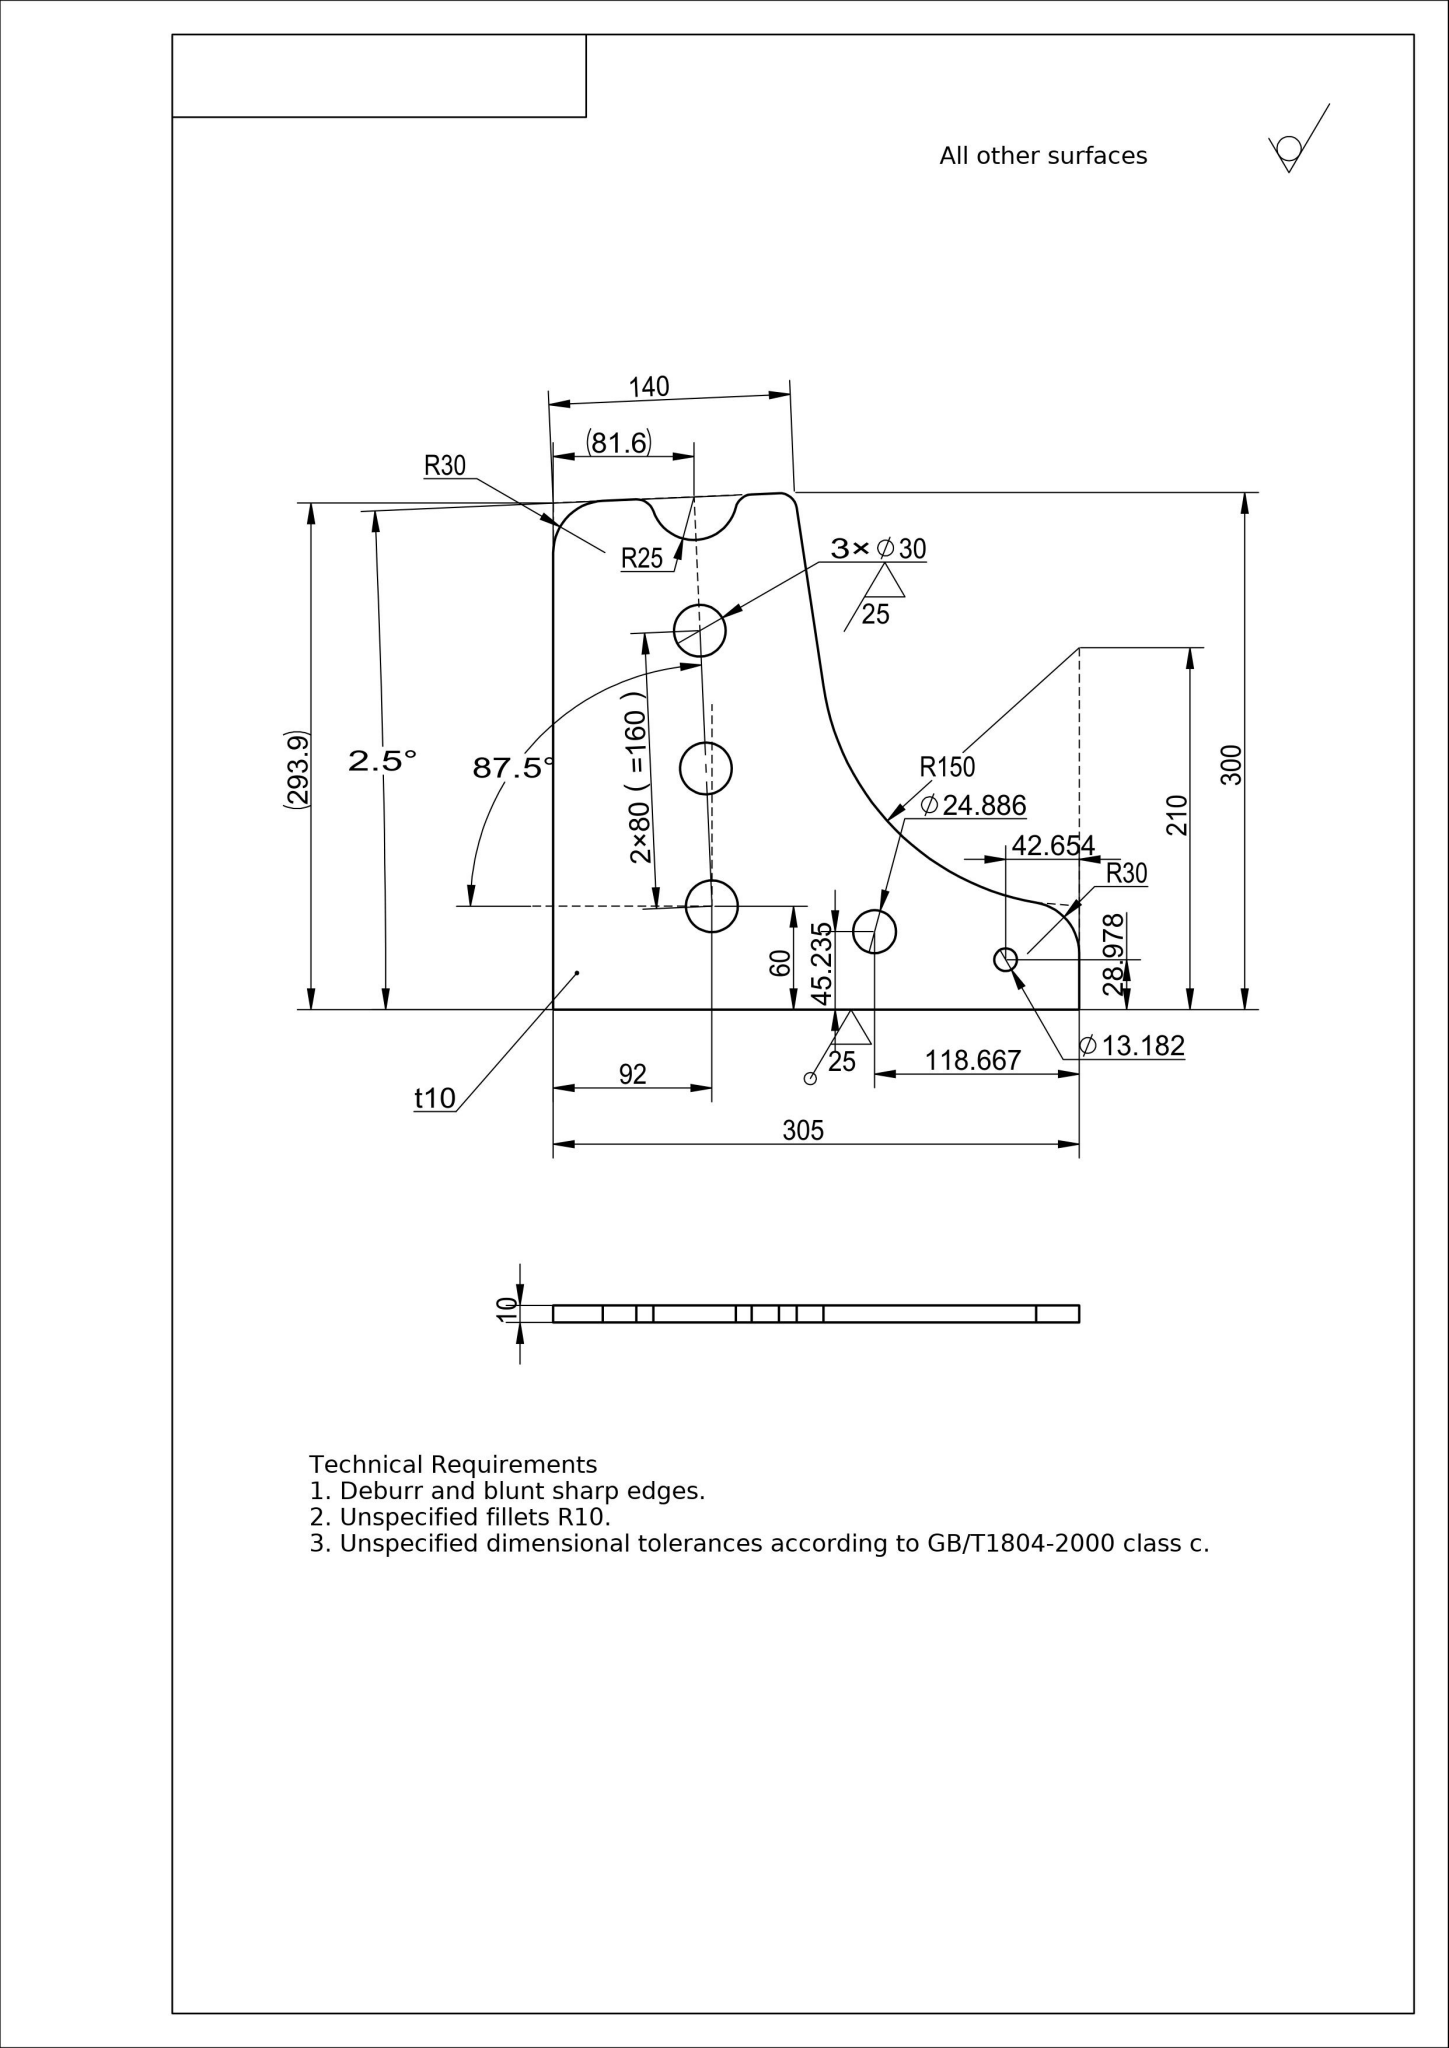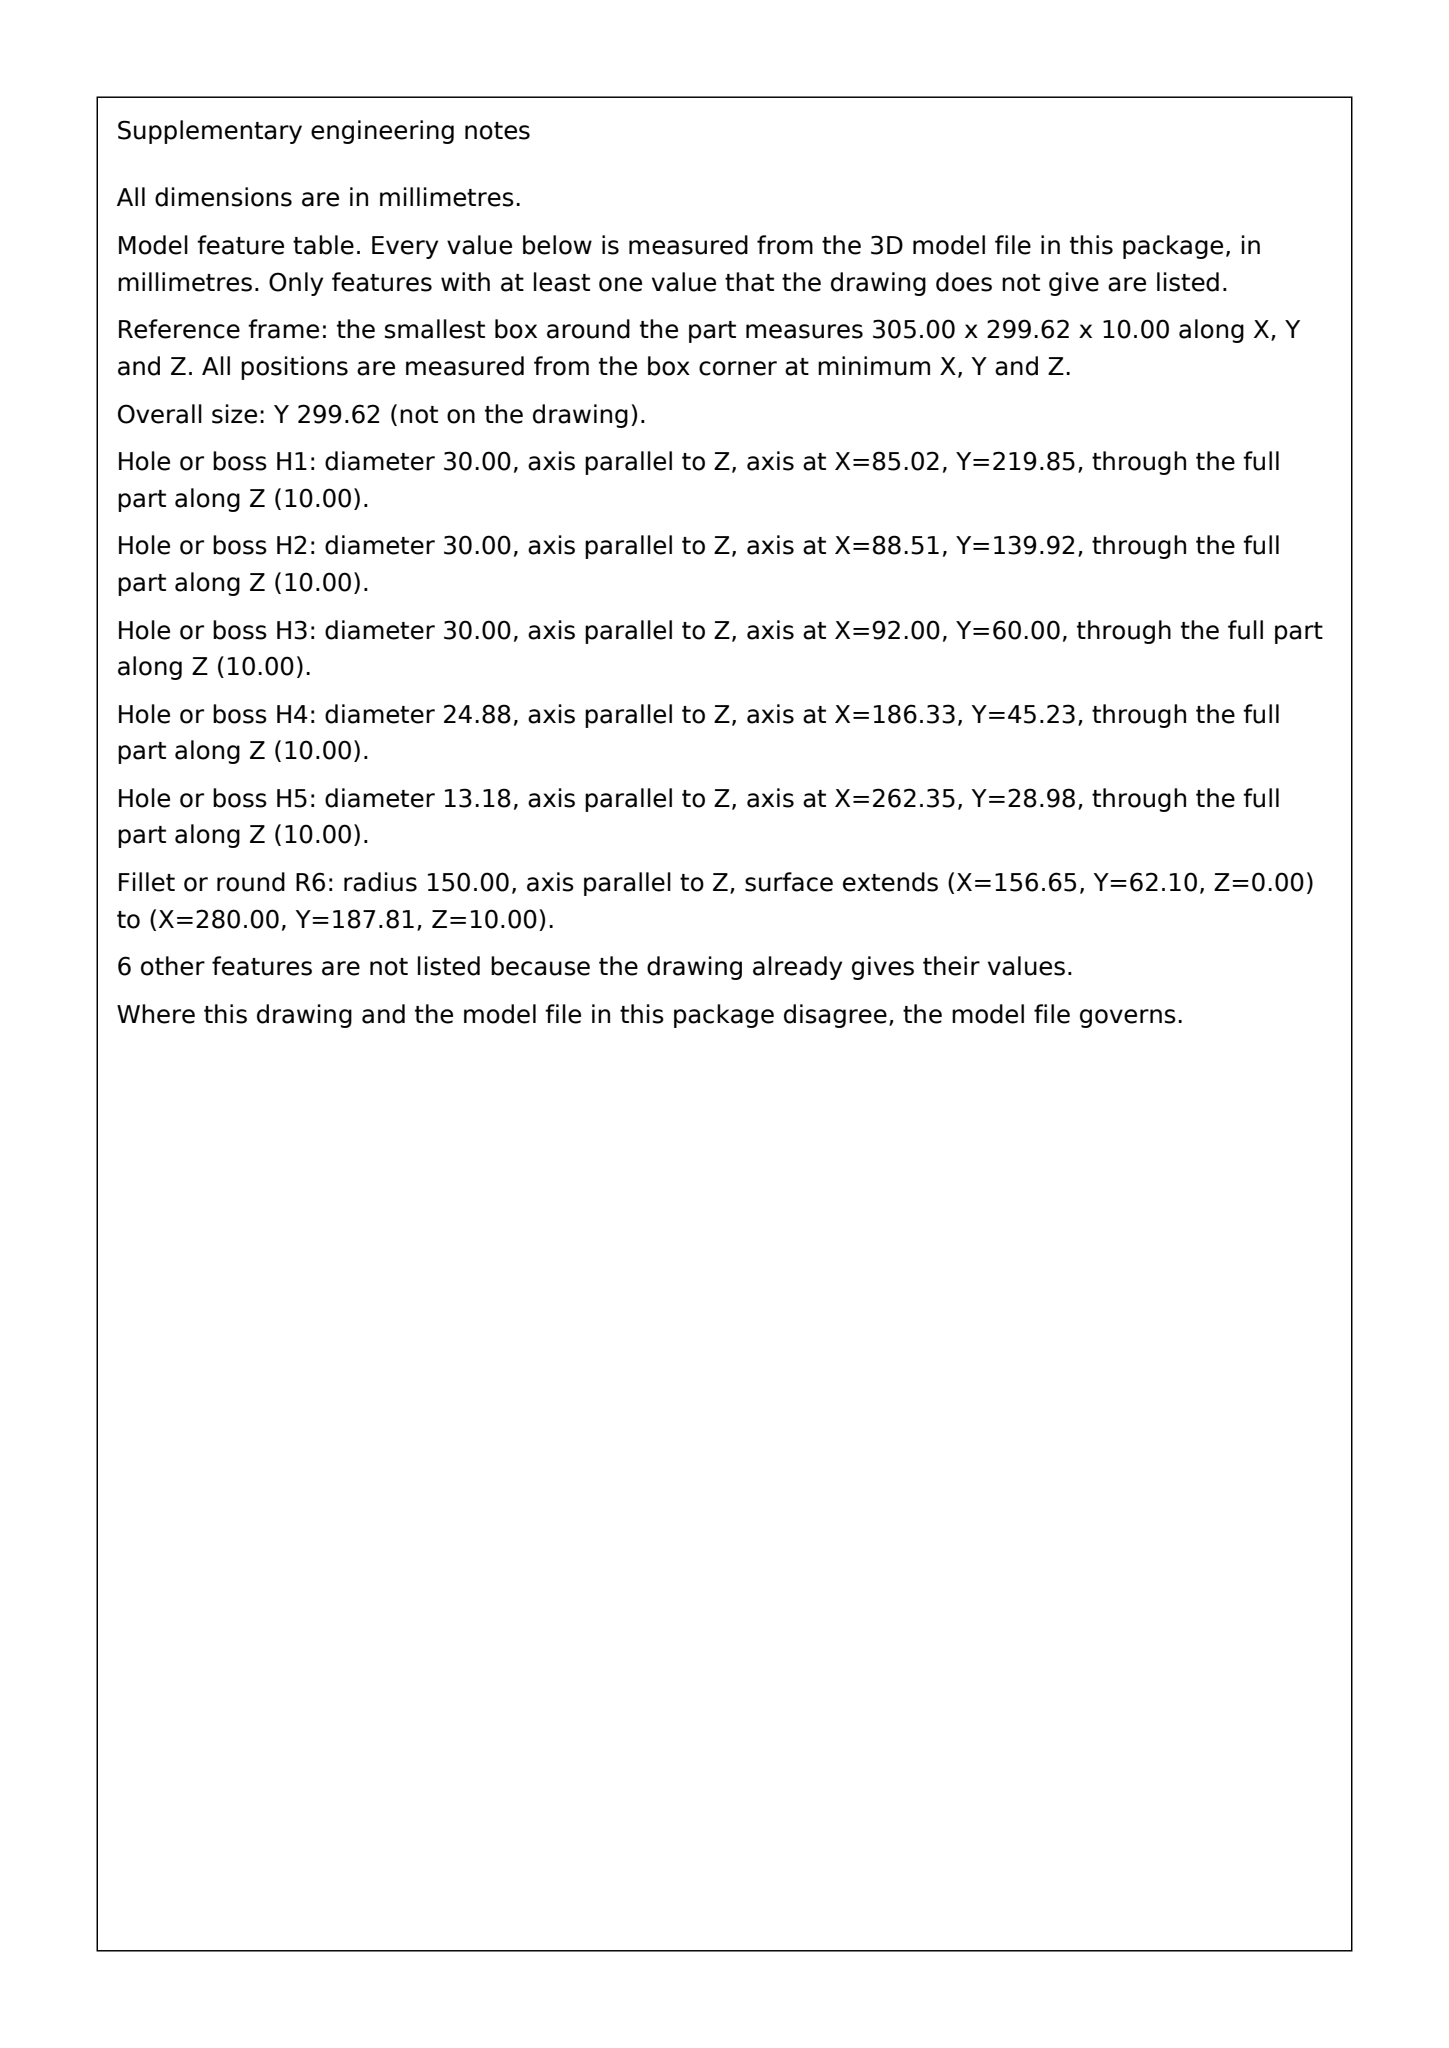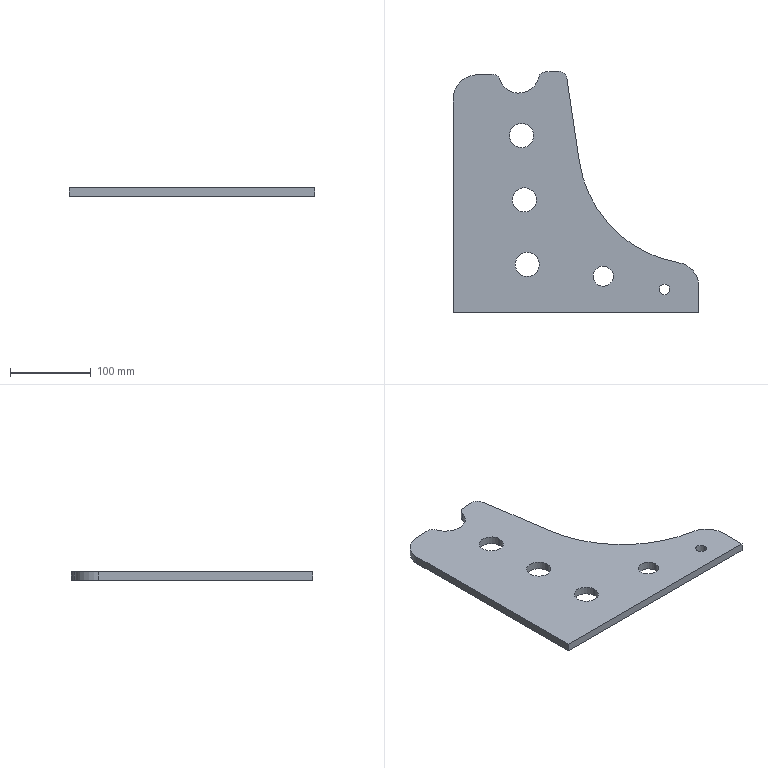Part | SolidWorks | mm | 1 solid | 25 faces | box 305 x 299.62 x 10 mm | volume 550435 mm3 | cylinder 17 | plane 8 | commonest cylinder face diameters 30 x6 20 x3 24.886 x2 13.182 x2 60 x2 50 x1 300 x1
STEP:
#1=CARTESIAN_POINT('',(198.776,45.235,-10.));
#2=VERTEX_POINT('',#1);
#3=CARTESIAN_POINT('',(173.889,45.235,-10.));
#4=VERTEX_POINT('',#3);
#5=CARTESIAN_POINT('',(186.333,45.235,-10.));
#6=DIRECTION('',(0.,0.,-1.));
#7=DIRECTION('',(-1.,0.,0.));
#8=AXIS2_PLACEMENT_3D('',#5,#6,#7);
#9=CIRCLE('',#8,12.443);
#10=EDGE_CURVE('',#2,#4,#9,.T.);
#11=ORIENTED_EDGE('',*,*,#10,.T.);
#12=CARTESIAN_POINT('',(173.889,45.235,0.));
#13=VERTEX_POINT('',#12);
#14=CARTESIAN_POINT('',(173.889,45.235,-70.));
#15=DIRECTION('',(0.,0.,1.));
#16=VECTOR('',#15,1000.);
#17=LINE('',#14,#16);
#18=EDGE_CURVE('',#4,#13,#17,.T.);
#19=ORIENTED_EDGE('',*,*,#18,.T.);
#20=CARTESIAN_POINT('',(198.776,45.235,0.));
#21=VERTEX_POINT('',#20);
#22=CARTESIAN_POINT('',(186.333,45.235,0.));
#23=DIRECTION('',(0.,0.,1.));
#24=DIRECTION('',(1.,0.,0.));
#25=AXIS2_PLACEMENT_3D('',#22,#23,#24);
#26=CIRCLE('',#25,12.443);
#27=EDGE_CURVE('',#13,#21,#26,.T.);
#28=ORIENTED_EDGE('',*,*,#27,.T.);
#29=CARTESIAN_POINT('',(198.776,45.235,-70.));
#30=DIRECTION('',(0.,0.,1.));
#31=VECTOR('',#30,1000.);
#32=LINE('',#29,#31);
#33=EDGE_CURVE('',#2,#21,#32,.T.);
#34=ORIENTED_EDGE('',*,*,#33,.F.);
#35=EDGE_LOOP('',(#11,#19,#28,#34));
#36=FACE_OUTER_BOUND('',#35,.T.);
#37=CARTESIAN_POINT('',(186.333,45.235,-70.));
#38=DIRECTION('',(0.,0.,1.));
#39=DIRECTION('',(1.,0.,0.));
#40=AXIS2_PLACEMENT_3D('',#37,#38,#39);
#41=CYLINDRICAL_SURFACE('',#40,12.443);
#42=ADVANCED_FACE('',(#36),#41,.F.);
#43=CARTESIAN_POINT('',(268.937,28.978,-10.));
#44=VERTEX_POINT('',#43);
#45=CARTESIAN_POINT('',(255.755,28.978,-10.));
#46=VERTEX_POINT('',#45);
#47=CARTESIAN_POINT('',(262.346,28.978,-10.));
#48=DIRECTION('',(0.,0.,-1.));
#49=DIRECTION('',(-1.,0.,0.));
#50=AXIS2_PLACEMENT_3D('',#47,#48,#49);
#51=CIRCLE('',#50,6.591);
#52=EDGE_CURVE('',#44,#46,#51,.T.);
#53=ORIENTED_EDGE('',*,*,#52,.T.);
#54=CARTESIAN_POINT('',(255.755,28.978,0.));
#55=VERTEX_POINT('',#54);
#56=CARTESIAN_POINT('',(255.755,28.978,-70.));
#57=DIRECTION('',(0.,0.,1.));
#58=VECTOR('',#57,1000.);
#59=LINE('',#56,#58);
#60=EDGE_CURVE('',#46,#55,#59,.T.);
#61=ORIENTED_EDGE('',*,*,#60,.T.);
#62=CARTESIAN_POINT('',(268.937,28.978,0.));
#63=VERTEX_POINT('',#62);
#64=CARTESIAN_POINT('',(262.346,28.978,0.));
#65=DIRECTION('',(0.,0.,1.));
#66=DIRECTION('',(1.,0.,0.));
#67=AXIS2_PLACEMENT_3D('',#64,#65,#66);
#68=CIRCLE('',#67,6.591);
#69=EDGE_CURVE('',#55,#63,#68,.T.);
#70=ORIENTED_EDGE('',*,*,#69,.T.);
#71=CARTESIAN_POINT('',(268.937,28.978,-70.));
#72=DIRECTION('',(0.,0.,1.));
#73=VECTOR('',#72,1000.);
#74=LINE('',#71,#73);
#75=EDGE_CURVE('',#44,#63,#74,.T.);
#76=ORIENTED_EDGE('',*,*,#75,.F.);
#77=EDGE_LOOP('',(#53,#61,#70,#76));
#78=FACE_OUTER_BOUND('',#77,.T.);
#79=CARTESIAN_POINT('',(262.346,28.978,-70.));
#80=DIRECTION('',(0.,0.,1.));
#81=DIRECTION('',(1.,0.,0.));
#82=AXIS2_PLACEMENT_3D('',#79,#80,#81);
#83=CYLINDRICAL_SURFACE('',#82,6.591);
#84=ADVANCED_FACE('',(#78),#83,.F.);
#85=CARTESIAN_POINT('',(77.,60.,-10.));
#86=VERTEX_POINT('',#85);
#87=CARTESIAN_POINT('',(107.,60.,-10.));
#88=VERTEX_POINT('',#87);
#89=CARTESIAN_POINT('',(92.,60.,-10.));
#90=DIRECTION('',(0.,0.,1.));
#91=DIRECTION('',(1.,0.,0.));
#92=AXIS2_PLACEMENT_3D('',#89,#90,#91);
#93=CIRCLE('',#92,15.);
#94=EDGE_CURVE('',#86,#88,#93,.T.);
#95=ORIENTED_EDGE('',*,*,#94,.F.);
#96=CARTESIAN_POINT('',(77.,60.,0.));
#97=VERTEX_POINT('',#96);
#98=CARTESIAN_POINT('',(77.,60.,-10.));
#99=DIRECTION('',(0.,0.,1.));
#100=VECTOR('',#99,1000.);
#101=LINE('',#98,#100);
#102=EDGE_CURVE('',#86,#97,#101,.T.);
#103=ORIENTED_EDGE('',*,*,#102,.T.);
#104=CARTESIAN_POINT('',(107.,60.,0.));
#105=VERTEX_POINT('',#104);
#106=CARTESIAN_POINT('',(92.,60.,0.));
#107=DIRECTION('',(0.,0.,1.));
#108=DIRECTION('',(1.,0.,0.));
#109=AXIS2_PLACEMENT_3D('',#106,#107,#108);
#110=CIRCLE('',#109,15.);
#111=EDGE_CURVE('',#97,#105,#110,.T.);
#112=ORIENTED_EDGE('',*,*,#111,.T.);
#113=CARTESIAN_POINT('',(107.,60.,-10.));
#114=DIRECTION('',(0.,0.,1.));
#115=VECTOR('',#114,1000.);
#116=LINE('',#113,#115);
#117=EDGE_CURVE('',#88,#105,#116,.T.);
#118=ORIENTED_EDGE('',*,*,#117,.F.);
#119=EDGE_LOOP('',(#95,#103,#112,#118));
#120=FACE_OUTER_BOUND('',#119,.T.);
#121=CARTESIAN_POINT('',(92.,60.,-10.));
#122=DIRECTION('',(0.,0.,1.));
#123=DIRECTION('',(1.,0.,0.));
#124=AXIS2_PLACEMENT_3D('',#121,#122,#123);
#125=CYLINDRICAL_SURFACE('',#124,15.);
#126=ADVANCED_FACE('',(#120),#125,.F.);
#127=CARTESIAN_POINT('',(73.51,139.924,-10.));
#128=VERTEX_POINT('',#127);
#129=CARTESIAN_POINT('',(103.51,139.924,-10.));
#130=VERTEX_POINT('',#129);
#131=CARTESIAN_POINT('',(88.51,139.924,-10.));
#132=DIRECTION('',(0.,0.,1.));
#133=DIRECTION('',(1.,0.,0.));
#134=AXIS2_PLACEMENT_3D('',#131,#132,#133);
#135=CIRCLE('',#134,15.);
#136=EDGE_CURVE('',#128,#130,#135,.T.);
#137=ORIENTED_EDGE('',*,*,#136,.F.);
#138=CARTESIAN_POINT('',(73.51,139.924,0.));
#139=VERTEX_POINT('',#138);
#140=CARTESIAN_POINT('',(73.51,139.924,-10.));
#141=DIRECTION('',(0.,0.,1.));
#142=VECTOR('',#141,1000.);
#143=LINE('',#140,#142);
#144=EDGE_CURVE('',#128,#139,#143,.T.);
#145=ORIENTED_EDGE('',*,*,#144,.T.);
#146=CARTESIAN_POINT('',(103.51,139.924,0.));
#147=VERTEX_POINT('',#146);
#148=CARTESIAN_POINT('',(88.51,139.924,0.));
#149=DIRECTION('',(0.,0.,1.));
#150=DIRECTION('',(1.,0.,0.));
#151=AXIS2_PLACEMENT_3D('',#148,#149,#150);
#152=CIRCLE('',#151,15.);
#153=EDGE_CURVE('',#139,#147,#152,.T.);
#154=ORIENTED_EDGE('',*,*,#153,.T.);
#155=CARTESIAN_POINT('',(103.51,139.924,-10.));
#156=DIRECTION('',(0.,0.,1.));
#157=VECTOR('',#156,1000.);
#158=LINE('',#155,#157);
#159=EDGE_CURVE('',#130,#147,#158,.T.);
#160=ORIENTED_EDGE('',*,*,#159,.F.);
#161=EDGE_LOOP('',(#137,#145,#154,#160));
#162=FACE_OUTER_BOUND('',#161,.T.);
#163=CARTESIAN_POINT('',(88.51,139.924,-10.));
#164=DIRECTION('',(0.,0.,1.));
#165=DIRECTION('',(1.,0.,0.));
#166=AXIS2_PLACEMENT_3D('',#163,#164,#165);
#167=CYLINDRICAL_SURFACE('',#166,15.);
#168=ADVANCED_FACE('',(#162),#167,.F.);
#169=CARTESIAN_POINT('',(70.021,219.848,-10.));
#170=VERTEX_POINT('',#169);
#171=CARTESIAN_POINT('',(100.021,219.848,-10.));
#172=VERTEX_POINT('',#171);
#173=CARTESIAN_POINT('',(85.021,219.848,-10.));
#174=DIRECTION('',(0.,0.,1.));
#175=DIRECTION('',(1.,0.,0.));
#176=AXIS2_PLACEMENT_3D('',#173,#174,#175);
#177=CIRCLE('',#176,15.);
#178=EDGE_CURVE('',#170,#172,#177,.T.);
#179=ORIENTED_EDGE('',*,*,#178,.F.);
#180=CARTESIAN_POINT('',(70.021,219.848,0.));
#181=VERTEX_POINT('',#180);
#182=CARTESIAN_POINT('',(70.021,219.848,-10.));
#183=DIRECTION('',(0.,0.,1.));
#184=VECTOR('',#183,1000.);
#185=LINE('',#182,#184);
#186=EDGE_CURVE('',#170,#181,#185,.T.);
#187=ORIENTED_EDGE('',*,*,#186,.T.);
#188=CARTESIAN_POINT('',(100.021,219.848,0.));
#189=VERTEX_POINT('',#188);
#190=CARTESIAN_POINT('',(85.021,219.848,0.));
#191=DIRECTION('',(0.,0.,1.));
#192=DIRECTION('',(1.,0.,0.));
#193=AXIS2_PLACEMENT_3D('',#190,#191,#192);
#194=CIRCLE('',#193,15.);
#195=EDGE_CURVE('',#181,#189,#194,.T.);
#196=ORIENTED_EDGE('',*,*,#195,.T.);
#197=CARTESIAN_POINT('',(100.021,219.848,-10.));
#198=DIRECTION('',(0.,0.,1.));
#199=VECTOR('',#198,1000.);
#200=LINE('',#197,#199);
#201=EDGE_CURVE('',#172,#189,#200,.T.);
#202=ORIENTED_EDGE('',*,*,#201,.F.);
#203=EDGE_LOOP('',(#179,#187,#196,#202));
#204=FACE_OUTER_BOUND('',#203,.T.);
#205=CARTESIAN_POINT('',(85.021,219.848,-10.));
#206=DIRECTION('',(0.,0.,1.));
#207=DIRECTION('',(1.,0.,0.));
#208=AXIS2_PLACEMENT_3D('',#205,#206,#207);
#209=CYLINDRICAL_SURFACE('',#208,15.);
#210=ADVANCED_FACE('',(#204),#209,.F.);
#211=CARTESIAN_POINT('',(0.,0.,0.));
#212=VERTEX_POINT('',#211);
#213=CARTESIAN_POINT('',(305.,0.,0.));
#214=VERTEX_POINT('',#213);
#215=CARTESIAN_POINT('',(0.,0.,0.));
#216=DIRECTION('',(1.,0.,0.));
#217=VECTOR('',#216,1000.);
#218=LINE('',#215,#217);
#219=EDGE_CURVE('',#212,#214,#218,.T.);
#220=ORIENTED_EDGE('',*,*,#219,.F.);
#221=CARTESIAN_POINT('',(0.,0.,-10.));
#222=VERTEX_POINT('',#221);
#223=CARTESIAN_POINT('',(0.,0.,-10.));
#224=DIRECTION('',(0.,0.,1.));
#225=VECTOR('',#224,1000.);
#226=LINE('',#223,#225);
#227=EDGE_CURVE('',#222,#212,#226,.T.);
#228=ORIENTED_EDGE('',*,*,#227,.F.);
#229=CARTESIAN_POINT('',(305.,0.,-10.));
#230=VERTEX_POINT('',#229);
#231=CARTESIAN_POINT('',(0.,0.,-10.));
#232=DIRECTION('',(1.,0.,0.));
#233=VECTOR('',#232,1000.);
#234=LINE('',#231,#233);
#235=EDGE_CURVE('',#222,#230,#234,.T.);
#236=ORIENTED_EDGE('',*,*,#235,.T.);
#237=CARTESIAN_POINT('',(305.,0.,-10.));
#238=DIRECTION('',(0.,0.,1.));
#239=VECTOR('',#238,1000.);
#240=LINE('',#237,#239);
#241=EDGE_CURVE('',#230,#214,#240,.T.);
#242=ORIENTED_EDGE('',*,*,#241,.T.);
#243=EDGE_LOOP('',(#220,#228,#236,#242));
#244=FACE_OUTER_BOUND('',#243,.T.);
#245=CARTESIAN_POINT('',(0.,0.,-10.));
#246=DIRECTION('',(0.,-1.,0.));
#247=DIRECTION('',(0.,0.,-1.));
#248=AXIS2_PLACEMENT_3D('',#245,#246,#247);
#249=PLANE('',#248);
#250=ADVANCED_FACE('',(#244),#249,.T.);
#251=CARTESIAN_POINT('',(-0.,265.175,0.));
#252=VERTEX_POINT('',#251);
#253=CARTESIAN_POINT('',(-0.,293.893,0.));
#254=DIRECTION('',(0.,-1.,0.));
#255=VECTOR('',#254,1000.);
#256=LINE('',#253,#255);
#257=EDGE_CURVE('',#252,#212,#256,.T.);
#258=ORIENTED_EDGE('',*,*,#257,.F.);
#259=CARTESIAN_POINT('',(-0.,265.175,-10.));
#260=VERTEX_POINT('',#259);
#261=CARTESIAN_POINT('',(-0.,265.175,-10.));
#262=DIRECTION('',(0.,0.,-1.));
#263=VECTOR('',#262,1000.);
#264=LINE('',#261,#263);
#265=EDGE_CURVE('',#252,#260,#264,.T.);
#266=ORIENTED_EDGE('',*,*,#265,.T.);
#267=CARTESIAN_POINT('',(-0.,293.893,-10.));
#268=DIRECTION('',(0.,-1.,0.));
#269=VECTOR('',#268,1000.);
#270=LINE('',#267,#269);
#271=EDGE_CURVE('',#260,#222,#270,.T.);
#272=ORIENTED_EDGE('',*,*,#271,.T.);
#273=ORIENTED_EDGE('',*,*,#227,.T.);
#274=EDGE_LOOP('',(#258,#266,#272,#273));
#275=FACE_OUTER_BOUND('',#274,.T.);
#276=CARTESIAN_POINT('',(-0.,293.893,-10.));
#277=DIRECTION('',(-1.,-0.,0.));
#278=DIRECTION('',(0.,-1.,0.));
#279=AXIS2_PLACEMENT_3D('',#276,#277,#278);
#280=PLANE('',#279);
#281=ADVANCED_FACE('',(#275),#280,.T.);
#282=CARTESIAN_POINT('',(48.123,295.994,-10.));
#283=VERTEX_POINT('',#282);
#284=CARTESIAN_POINT('',(28.691,295.146,-10.));
#285=VERTEX_POINT('',#284);
#286=CARTESIAN_POINT('',(56.656,296.367,-10.));
#287=DIRECTION('',(-0.999,-0.04362,0.));
#288=VECTOR('',#287,1000.);
#289=LINE('',#286,#288);
#290=EDGE_CURVE('',#283,#285,#289,.T.);
#291=ORIENTED_EDGE('',*,*,#290,.T.);
#292=CARTESIAN_POINT('',(28.691,295.146,0.));
#293=VERTEX_POINT('',#292);
#294=CARTESIAN_POINT('',(28.691,295.146,-10.));
#295=DIRECTION('',(0.,0.,1.));
#296=VECTOR('',#295,1000.);
#297=LINE('',#294,#296);
#298=EDGE_CURVE('',#285,#293,#297,.T.);
#299=ORIENTED_EDGE('',*,*,#298,.T.);
#300=CARTESIAN_POINT('',(48.123,295.994,0.));
#301=VERTEX_POINT('',#300);
#302=CARTESIAN_POINT('',(56.656,296.367,0.));
#303=DIRECTION('',(-0.999,-0.04362,0.));
#304=VECTOR('',#303,1000.);
#305=LINE('',#302,#304);
#306=EDGE_CURVE('',#301,#293,#305,.T.);
#307=ORIENTED_EDGE('',*,*,#306,.F.);
#308=CARTESIAN_POINT('',(48.123,295.994,-10.));
#309=DIRECTION('',(0.,0.,-1.));
#310=VECTOR('',#309,1000.);
#311=LINE('',#308,#310);
#312=EDGE_CURVE('',#301,#283,#311,.T.);
#313=ORIENTED_EDGE('',*,*,#312,.T.);
#314=EDGE_LOOP('',(#291,#299,#307,#313));
#315=FACE_OUTER_BOUND('',#314,.T.);
#316=CARTESIAN_POINT('',(56.656,296.367,-10.));
#317=DIRECTION('',(-0.04362,0.999,0.));
#318=DIRECTION('',(-0.999,-0.04362,0.));
#319=AXIS2_PLACEMENT_3D('',#316,#317,#318);
#320=PLANE('',#319);
#321=ADVANCED_FACE('',(#315),#320,.T.);
#322=CARTESIAN_POINT('',(105.879,291.366,-10.));
#323=VERTEX_POINT('',#322);
#324=CARTESIAN_POINT('',(58.009,289.276,-10.));
#325=VERTEX_POINT('',#324);
#326=CARTESIAN_POINT('',(81.632,297.457,-10.));
#327=DIRECTION('',(0.,0.,-1.));
#328=DIRECTION('',(1.,0.,0.));
#329=AXIS2_PLACEMENT_3D('',#326,#327,#328);
#330=CIRCLE('',#329,25.);
#331=EDGE_CURVE('',#323,#325,#330,.T.);
#332=ORIENTED_EDGE('',*,*,#331,.T.);
#333=CARTESIAN_POINT('',(58.009,289.276,0.));
#334=VERTEX_POINT('',#333);
#335=CARTESIAN_POINT('',(58.009,289.276,-10.));
#336=DIRECTION('',(0.,0.,1.));
#337=VECTOR('',#336,1000.);
#338=LINE('',#335,#337);
#339=EDGE_CURVE('',#325,#334,#338,.T.);
#340=ORIENTED_EDGE('',*,*,#339,.T.);
#341=CARTESIAN_POINT('',(105.879,291.366,0.));
#342=VERTEX_POINT('',#341);
#343=CARTESIAN_POINT('',(81.632,297.457,0.));
#344=DIRECTION('',(0.,0.,-1.));
#345=DIRECTION('',(1.,0.,0.));
#346=AXIS2_PLACEMENT_3D('',#343,#344,#345);
#347=CIRCLE('',#346,25.);
#348=EDGE_CURVE('',#342,#334,#347,.T.);
#349=ORIENTED_EDGE('',*,*,#348,.F.);
#350=CARTESIAN_POINT('',(105.879,291.366,-10.));
#351=DIRECTION('',(0.,0.,-1.));
#352=VECTOR('',#351,1000.);
#353=LINE('',#350,#352);
#354=EDGE_CURVE('',#342,#323,#353,.T.);
#355=ORIENTED_EDGE('',*,*,#354,.T.);
#356=EDGE_LOOP('',(#332,#340,#349,#355));
#357=FACE_OUTER_BOUND('',#356,.T.);
#358=CARTESIAN_POINT('',(81.632,297.457,-10.));
#359=DIRECTION('',(0.,0.,1.));
#360=DIRECTION('',(1.,0.,0.));
#361=AXIS2_PLACEMENT_3D('',#358,#359,#360);
#362=CYLINDRICAL_SURFACE('',#361,25.);
#363=ADVANCED_FACE('',(#357),#362,.F.);
#364=CARTESIAN_POINT('',(130.873,299.607,0.));
#365=VERTEX_POINT('',#364);
#366=CARTESIAN_POINT('',(115.141,298.92,0.));
#367=VERTEX_POINT('',#366);
#368=CARTESIAN_POINT('',(139.867,300.,0.));
#369=DIRECTION('',(-0.999,-0.04362,0.));
#370=VECTOR('',#369,1000.);
#371=LINE('',#368,#370);
#372=EDGE_CURVE('',#365,#367,#371,.T.);
#373=ORIENTED_EDGE('',*,*,#372,.F.);
#374=CARTESIAN_POINT('',(130.873,299.607,-10.));
#375=VERTEX_POINT('',#374);
#376=CARTESIAN_POINT('',(130.873,299.607,-10.));
#377=DIRECTION('',(0.,0.,-1.));
#378=VECTOR('',#377,1000.);
#379=LINE('',#376,#378);
#380=EDGE_CURVE('',#365,#375,#379,.T.);
#381=ORIENTED_EDGE('',*,*,#380,.T.);
#382=CARTESIAN_POINT('',(115.141,298.92,-10.));
#383=VERTEX_POINT('',#382);
#384=CARTESIAN_POINT('',(139.867,300.,-10.));
#385=DIRECTION('',(-0.999,-0.04362,0.));
#386=VECTOR('',#385,1000.);
#387=LINE('',#384,#386);
#388=EDGE_CURVE('',#375,#383,#387,.T.);
#389=ORIENTED_EDGE('',*,*,#388,.T.);
#390=CARTESIAN_POINT('',(115.141,298.92,-10.));
#391=DIRECTION('',(0.,0.,1.));
#392=VECTOR('',#391,1000.);
#393=LINE('',#390,#392);
#394=EDGE_CURVE('',#383,#367,#393,.T.);
#395=ORIENTED_EDGE('',*,*,#394,.T.);
#396=EDGE_LOOP('',(#373,#381,#389,#395));
#397=FACE_OUTER_BOUND('',#396,.T.);
#398=CARTESIAN_POINT('',(139.867,300.,-10.));
#399=DIRECTION('',(-0.04362,0.999,0.));
#400=DIRECTION('',(-0.999,-0.04362,0.));
#401=AXIS2_PLACEMENT_3D('',#398,#399,#400);
#402=PLANE('',#401);
#403=ADVANCED_FACE('',(#397),#402,.T.);
#404=CARTESIAN_POINT('',(156.651,187.807,-10.));
#405=VERTEX_POINT('',#404);
#406=CARTESIAN_POINT('',(141.199,291.096,-10.));
#407=VERTEX_POINT('',#406);
#408=CARTESIAN_POINT('',(156.651,187.807,-10.));
#409=DIRECTION('',(-0.148,0.989,0.));
#410=VECTOR('',#409,1000.);
#411=LINE('',#408,#410);
#412=EDGE_CURVE('',#405,#407,#411,.T.);
#413=ORIENTED_EDGE('',*,*,#412,.T.);
#414=CARTESIAN_POINT('',(141.199,291.096,0.));
#415=VERTEX_POINT('',#414);
#416=CARTESIAN_POINT('',(141.199,291.096,-10.));
#417=DIRECTION('',(0.,0.,1.));
#418=VECTOR('',#417,1000.);
#419=LINE('',#416,#418);
#420=EDGE_CURVE('',#407,#415,#419,.T.);
#421=ORIENTED_EDGE('',*,*,#420,.T.);
#422=CARTESIAN_POINT('',(156.651,187.807,0.));
#423=VERTEX_POINT('',#422);
#424=CARTESIAN_POINT('',(156.651,187.807,0.));
#425=DIRECTION('',(-0.148,0.989,0.));
#426=VECTOR('',#425,1000.);
#427=LINE('',#424,#426);
#428=EDGE_CURVE('',#423,#415,#427,.T.);
#429=ORIENTED_EDGE('',*,*,#428,.F.);
#430=CARTESIAN_POINT('',(156.651,187.807,-10.));
#431=DIRECTION('',(0.,0.,1.));
#432=VECTOR('',#431,1000.);
#433=LINE('',#430,#432);
#434=EDGE_CURVE('',#405,#423,#433,.T.);
#435=ORIENTED_EDGE('',*,*,#434,.F.);
#436=EDGE_LOOP('',(#413,#421,#429,#435));
#437=FACE_OUTER_BOUND('',#436,.T.);
#438=CARTESIAN_POINT('',(156.651,187.807,-10.));
#439=DIRECTION('',(0.989,0.148,0.));
#440=DIRECTION('',(-0.148,0.989,0.));
#441=AXIS2_PLACEMENT_3D('',#438,#439,#440);
#442=PLANE('',#441);
#443=ADVANCED_FACE('',(#437),#442,.T.);
#444=CARTESIAN_POINT('',(280.,62.098,0.));
#445=VERTEX_POINT('',#444);
#446=CARTESIAN_POINT('',(305.,210.,0.));
#447=DIRECTION('',(0.,0.,-1.));
#448=DIRECTION('',(-1.,0.,0.));
#449=AXIS2_PLACEMENT_3D('',#446,#447,#448);
#450=CIRCLE('',#449,150.);
#451=EDGE_CURVE('',#445,#423,#450,.T.);
#452=ORIENTED_EDGE('',*,*,#451,.F.);
#453=CARTESIAN_POINT('',(280.,62.098,-10.));
#454=VERTEX_POINT('',#453);
#455=CARTESIAN_POINT('',(280.,62.098,-10.));
#456=DIRECTION('',(0.,0.,-1.));
#457=VECTOR('',#456,1000.);
#458=LINE('',#455,#457);
#459=EDGE_CURVE('',#445,#454,#458,.T.);
#460=ORIENTED_EDGE('',*,*,#459,.T.);
#461=CARTESIAN_POINT('',(305.,210.,-10.));
#462=DIRECTION('',(0.,0.,-1.));
#463=DIRECTION('',(-1.,0.,0.));
#464=AXIS2_PLACEMENT_3D('',#461,#462,#463);
#465=CIRCLE('',#464,150.);
#466=EDGE_CURVE('',#454,#405,#465,.T.);
#467=ORIENTED_EDGE('',*,*,#466,.T.);
#468=ORIENTED_EDGE('',*,*,#434,.T.);
#469=EDGE_LOOP('',(#452,#460,#467,#468));
#470=FACE_OUTER_BOUND('',#469,.T.);
#471=CARTESIAN_POINT('',(305.,210.,-10.));
#472=DIRECTION('',(0.,0.,1.));
#473=DIRECTION('',(1.,0.,0.));
#474=AXIS2_PLACEMENT_3D('',#471,#472,#473);
#475=CYLINDRICAL_SURFACE('',#474,150.);
#476=ADVANCED_FACE('',(#470),#475,.F.);
#477=CARTESIAN_POINT('',(305.,32.518,-10.));
#478=VERTEX_POINT('',#477);
#479=CARTESIAN_POINT('',(305.,0.,-10.));
#480=DIRECTION('',(0.,1.,0.));
#481=VECTOR('',#480,1000.);
#482=LINE('',#479,#481);
#483=EDGE_CURVE('',#230,#478,#482,.T.);
#484=ORIENTED_EDGE('',*,*,#483,.T.);
#485=CARTESIAN_POINT('',(305.,32.518,0.));
#486=VERTEX_POINT('',#485);
#487=CARTESIAN_POINT('',(305.,32.518,-10.));
#488=DIRECTION('',(0.,0.,1.));
#489=VECTOR('',#488,1000.);
#490=LINE('',#487,#489);
#491=EDGE_CURVE('',#478,#486,#490,.T.);
#492=ORIENTED_EDGE('',*,*,#491,.T.);
#493=CARTESIAN_POINT('',(305.,0.,0.));
#494=DIRECTION('',(0.,1.,0.));
#495=VECTOR('',#494,1000.);
#496=LINE('',#493,#495);
#497=EDGE_CURVE('',#214,#486,#496,.T.);
#498=ORIENTED_EDGE('',*,*,#497,.F.);
#499=ORIENTED_EDGE('',*,*,#241,.F.);
#500=EDGE_LOOP('',(#484,#492,#498,#499));
#501=FACE_OUTER_BOUND('',#500,.T.);
#502=CARTESIAN_POINT('',(305.,0.,-10.));
#503=DIRECTION('',(1.,0.,0.));
#504=DIRECTION('',(0.,0.,-1.));
#505=AXIS2_PLACEMENT_3D('',#502,#503,#504);
#506=PLANE('',#505);
#507=ADVANCED_FACE('',(#501),#506,.T.);
#508=ORIENTED_EDGE('',*,*,#10,.F.);
#509=CARTESIAN_POINT('',(186.333,45.235,-10.));
#510=DIRECTION('',(0.,0.,-1.));
#511=DIRECTION('',(-1.,0.,0.));
#512=AXIS2_PLACEMENT_3D('',#509,#510,#511);
#513=CIRCLE('',#512,12.443);
#514=EDGE_CURVE('',#4,#2,#513,.T.);
#515=ORIENTED_EDGE('',*,*,#514,.F.);
#516=EDGE_LOOP('',(#508,#515));
#517=FACE_BOUND('',#516,.T.);
#518=ORIENTED_EDGE('',*,*,#52,.F.);
#519=CARTESIAN_POINT('',(262.346,28.978,-10.));
#520=DIRECTION('',(0.,0.,-1.));
#521=DIRECTION('',(-1.,0.,0.));
#522=AXIS2_PLACEMENT_3D('',#519,#520,#521);
#523=CIRCLE('',#522,6.591);
#524=EDGE_CURVE('',#46,#44,#523,.T.);
#525=ORIENTED_EDGE('',*,*,#524,.F.);
#526=EDGE_LOOP('',(#518,#525));
#527=FACE_BOUND('',#526,.T.);
#528=CARTESIAN_POINT('',(92.,60.,-10.));
#529=DIRECTION('',(0.,0.,1.));
#530=DIRECTION('',(1.,0.,0.));
#531=AXIS2_PLACEMENT_3D('',#528,#529,#530);
#532=CIRCLE('',#531,15.);
#533=EDGE_CURVE('',#88,#86,#532,.T.);
#534=ORIENTED_EDGE('',*,*,#533,.T.);
#535=ORIENTED_EDGE('',*,*,#94,.T.);
#536=EDGE_LOOP('',(#534,#535));
#537=FACE_BOUND('',#536,.T.);
#538=CARTESIAN_POINT('',(88.51,139.924,-10.));
#539=DIRECTION('',(0.,0.,1.));
#540=DIRECTION('',(1.,0.,0.));
#541=AXIS2_PLACEMENT_3D('',#538,#539,#540);
#542=CIRCLE('',#541,15.);
#543=EDGE_CURVE('',#130,#128,#542,.T.);
#544=ORIENTED_EDGE('',*,*,#543,.T.);
#545=ORIENTED_EDGE('',*,*,#136,.T.);
#546=EDGE_LOOP('',(#544,#545));
#547=FACE_BOUND('',#546,.T.);
#548=CARTESIAN_POINT('',(85.021,219.848,-10.));
#549=DIRECTION('',(0.,0.,1.));
#550=DIRECTION('',(1.,0.,0.));
#551=AXIS2_PLACEMENT_3D('',#548,#549,#550);
#552=CIRCLE('',#551,15.);
#553=EDGE_CURVE('',#172,#170,#552,.T.);
#554=ORIENTED_EDGE('',*,*,#553,.T.);
#555=ORIENTED_EDGE('',*,*,#178,.T.);
#556=EDGE_LOOP('',(#554,#555));
#557=FACE_BOUND('',#556,.T.);
#558=ORIENTED_EDGE('',*,*,#271,.F.);
#559=CARTESIAN_POINT('',(30.,265.175,-10.));
#560=DIRECTION('',(0.,0.,-1.));
#561=DIRECTION('',(-1.,0.,0.));
#562=AXIS2_PLACEMENT_3D('',#559,#560,#561);
#563=CIRCLE('',#562,30.);
#564=EDGE_CURVE('',#260,#285,#563,.T.);
#565=ORIENTED_EDGE('',*,*,#564,.T.);
#566=ORIENTED_EDGE('',*,*,#290,.F.);
#567=CARTESIAN_POINT('',(48.559,286.004,-10.));
#568=DIRECTION('',(0.,0.,-1.));
#569=DIRECTION('',(-1.,0.,0.));
#570=AXIS2_PLACEMENT_3D('',#567,#568,#569);
#571=CIRCLE('',#570,10.);
#572=EDGE_CURVE('',#283,#325,#571,.T.);
#573=ORIENTED_EDGE('',*,*,#572,.T.);
#574=ORIENTED_EDGE('',*,*,#331,.F.);
#575=CARTESIAN_POINT('',(115.578,288.93,-10.));
#576=DIRECTION('',(0.,0.,-1.));
#577=DIRECTION('',(-1.,0.,0.));
#578=AXIS2_PLACEMENT_3D('',#575,#576,#577);
#579=CIRCLE('',#578,10.);
#580=EDGE_CURVE('',#323,#383,#579,.T.);
#581=ORIENTED_EDGE('',*,*,#580,.T.);
#582=ORIENTED_EDGE('',*,*,#388,.F.);
#583=CARTESIAN_POINT('',(131.309,289.617,-10.));
#584=DIRECTION('',(0.,0.,-1.));
#585=DIRECTION('',(-1.,0.,0.));
#586=AXIS2_PLACEMENT_3D('',#583,#584,#585);
#587=CIRCLE('',#586,10.);
#588=EDGE_CURVE('',#375,#407,#587,.T.);
#589=ORIENTED_EDGE('',*,*,#588,.T.);
#590=ORIENTED_EDGE('',*,*,#412,.F.);
#591=ORIENTED_EDGE('',*,*,#466,.F.);
#592=CARTESIAN_POINT('',(275.,32.518,-10.));
#593=DIRECTION('',(0.,0.,-1.));
#594=DIRECTION('',(-1.,0.,0.));
#595=AXIS2_PLACEMENT_3D('',#592,#593,#594);
#596=CIRCLE('',#595,30.);
#597=EDGE_CURVE('',#454,#478,#596,.T.);
#598=ORIENTED_EDGE('',*,*,#597,.T.);
#599=ORIENTED_EDGE('',*,*,#483,.F.);
#600=ORIENTED_EDGE('',*,*,#235,.F.);
#601=EDGE_LOOP('',(#558,#565,#566,#573,#574,#581,#582,#589,#590,#591,#598,#599,#600));
#602=FACE_OUTER_BOUND('',#601,.T.);
#603=CARTESIAN_POINT('',(305.,210.,-10.));
#604=DIRECTION('',(0.,0.,-1.));
#605=DIRECTION('',(-1.,0.,0.));
#606=AXIS2_PLACEMENT_3D('',#603,#604,#605);
#607=PLANE('',#606);
#608=ADVANCED_FACE('',(#517,#527,#537,#547,#557,#602),#607,.T.);
#609=CARTESIAN_POINT('',(186.333,45.235,0.));
#610=DIRECTION('',(0.,0.,1.));
#611=DIRECTION('',(1.,0.,0.));
#612=AXIS2_PLACEMENT_3D('',#609,#610,#611);
#613=CIRCLE('',#612,12.443);
#614=EDGE_CURVE('',#21,#13,#613,.T.);
#615=ORIENTED_EDGE('',*,*,#614,.F.);
#616=ORIENTED_EDGE('',*,*,#27,.F.);
#617=EDGE_LOOP('',(#615,#616));
#618=FACE_BOUND('',#617,.T.);
#619=CARTESIAN_POINT('',(262.346,28.978,0.));
#620=DIRECTION('',(0.,0.,1.));
#621=DIRECTION('',(1.,0.,0.));
#622=AXIS2_PLACEMENT_3D('',#619,#620,#621);
#623=CIRCLE('',#622,6.591);
#624=EDGE_CURVE('',#63,#55,#623,.T.);
#625=ORIENTED_EDGE('',*,*,#624,.F.);
#626=ORIENTED_EDGE('',*,*,#69,.F.);
#627=EDGE_LOOP('',(#625,#626));
#628=FACE_BOUND('',#627,.T.);
#629=CARTESIAN_POINT('',(92.,60.,0.));
#630=DIRECTION('',(0.,0.,1.));
#631=DIRECTION('',(1.,0.,0.));
#632=AXIS2_PLACEMENT_3D('',#629,#630,#631);
#633=CIRCLE('',#632,15.);
#634=EDGE_CURVE('',#105,#97,#633,.T.);
#635=ORIENTED_EDGE('',*,*,#634,.F.);
#636=ORIENTED_EDGE('',*,*,#111,.F.);
#637=EDGE_LOOP('',(#635,#636));
#638=FACE_BOUND('',#637,.T.);
#639=CARTESIAN_POINT('',(88.51,139.924,0.));
#640=DIRECTION('',(0.,0.,1.));
#641=DIRECTION('',(1.,0.,0.));
#642=AXIS2_PLACEMENT_3D('',#639,#640,#641);
#643=CIRCLE('',#642,15.);
#644=EDGE_CURVE('',#147,#139,#643,.T.);
#645=ORIENTED_EDGE('',*,*,#644,.F.);
#646=ORIENTED_EDGE('',*,*,#153,.F.);
#647=EDGE_LOOP('',(#645,#646));
#648=FACE_BOUND('',#647,.T.);
#649=CARTESIAN_POINT('',(85.021,219.848,0.));
#650=DIRECTION('',(0.,0.,1.));
#651=DIRECTION('',(1.,0.,0.));
#652=AXIS2_PLACEMENT_3D('',#649,#650,#651);
#653=CIRCLE('',#652,15.);
#654=EDGE_CURVE('',#189,#181,#653,.T.);
#655=ORIENTED_EDGE('',*,*,#654,.F.);
#656=ORIENTED_EDGE('',*,*,#195,.F.);
#657=EDGE_LOOP('',(#655,#656));
#658=FACE_BOUND('',#657,.T.);
#659=ORIENTED_EDGE('',*,*,#306,.T.);
#660=CARTESIAN_POINT('',(30.,265.175,0.));
#661=DIRECTION('',(0.,0.,1.));
#662=DIRECTION('',(-1.,0.,0.));
#663=AXIS2_PLACEMENT_3D('',#660,#661,#662);
#664=CIRCLE('',#663,30.);
#665=EDGE_CURVE('',#293,#252,#664,.T.);
#666=ORIENTED_EDGE('',*,*,#665,.T.);
#667=ORIENTED_EDGE('',*,*,#257,.T.);
#668=ORIENTED_EDGE('',*,*,#219,.T.);
#669=ORIENTED_EDGE('',*,*,#497,.T.);
#670=CARTESIAN_POINT('',(275.,32.518,0.));
#671=DIRECTION('',(0.,0.,1.));
#672=DIRECTION('',(-1.,0.,0.));
#673=AXIS2_PLACEMENT_3D('',#670,#671,#672);
#674=CIRCLE('',#673,30.);
#675=EDGE_CURVE('',#486,#445,#674,.T.);
#676=ORIENTED_EDGE('',*,*,#675,.T.);
#677=ORIENTED_EDGE('',*,*,#451,.T.);
#678=ORIENTED_EDGE('',*,*,#428,.T.);
#679=CARTESIAN_POINT('',(131.309,289.617,0.));
#680=DIRECTION('',(0.,0.,1.));
#681=DIRECTION('',(-1.,0.,0.));
#682=AXIS2_PLACEMENT_3D('',#679,#680,#681);
#683=CIRCLE('',#682,10.);
#684=EDGE_CURVE('',#415,#365,#683,.T.);
#685=ORIENTED_EDGE('',*,*,#684,.T.);
#686=ORIENTED_EDGE('',*,*,#372,.T.);
#687=CARTESIAN_POINT('',(115.578,288.93,0.));
#688=DIRECTION('',(0.,0.,1.));
#689=DIRECTION('',(-1.,0.,0.));
#690=AXIS2_PLACEMENT_3D('',#687,#688,#689);
#691=CIRCLE('',#690,10.);
#692=EDGE_CURVE('',#367,#342,#691,.T.);
#693=ORIENTED_EDGE('',*,*,#692,.T.);
#694=ORIENTED_EDGE('',*,*,#348,.T.);
#695=CARTESIAN_POINT('',(48.559,286.004,0.));
#696=DIRECTION('',(0.,0.,1.));
#697=DIRECTION('',(-1.,0.,0.));
#698=AXIS2_PLACEMENT_3D('',#695,#696,#697);
#699=CIRCLE('',#698,10.);
#700=EDGE_CURVE('',#334,#301,#699,.T.);
#701=ORIENTED_EDGE('',*,*,#700,.T.);
#702=EDGE_LOOP('',(#659,#666,#667,#668,#669,#676,#677,#678,#685,#686,#693,#694,#701));
#703=FACE_OUTER_BOUND('',#702,.T.);
#704=CARTESIAN_POINT('',(305.,210.,0.));
#705=DIRECTION('',(0.,0.,-1.));
#706=DIRECTION('',(-1.,0.,0.));
#707=AXIS2_PLACEMENT_3D('',#704,#705,#706);
#708=PLANE('',#707);
#709=ADVANCED_FACE('',(#618,#628,#638,#648,#658,#703),#708,.F.);
#710=ORIENTED_EDGE('',*,*,#186,.F.);
#711=ORIENTED_EDGE('',*,*,#553,.F.);
#712=ORIENTED_EDGE('',*,*,#201,.T.);
#713=ORIENTED_EDGE('',*,*,#654,.T.);
#714=EDGE_LOOP('',(#710,#711,#712,#713));
#715=FACE_OUTER_BOUND('',#714,.T.);
#716=CARTESIAN_POINT('',(85.021,219.848,-10.));
#717=DIRECTION('',(0.,0.,1.));
#718=DIRECTION('',(1.,0.,0.));
#719=AXIS2_PLACEMENT_3D('',#716,#717,#718);
#720=CYLINDRICAL_SURFACE('',#719,15.);
#721=ADVANCED_FACE('',(#715),#720,.F.);
#722=ORIENTED_EDGE('',*,*,#144,.F.);
#723=ORIENTED_EDGE('',*,*,#543,.F.);
#724=ORIENTED_EDGE('',*,*,#159,.T.);
#725=ORIENTED_EDGE('',*,*,#644,.T.);
#726=EDGE_LOOP('',(#722,#723,#724,#725));
#727=FACE_OUTER_BOUND('',#726,.T.);
#728=CARTESIAN_POINT('',(88.51,139.924,-10.));
#729=DIRECTION('',(0.,0.,1.));
#730=DIRECTION('',(1.,0.,0.));
#731=AXIS2_PLACEMENT_3D('',#728,#729,#730);
#732=CYLINDRICAL_SURFACE('',#731,15.);
#733=ADVANCED_FACE('',(#727),#732,.F.);
#734=ORIENTED_EDGE('',*,*,#102,.F.);
#735=ORIENTED_EDGE('',*,*,#533,.F.);
#736=ORIENTED_EDGE('',*,*,#117,.T.);
#737=ORIENTED_EDGE('',*,*,#634,.T.);
#738=EDGE_LOOP('',(#734,#735,#736,#737));
#739=FACE_OUTER_BOUND('',#738,.T.);
#740=CARTESIAN_POINT('',(92.,60.,-10.));
#741=DIRECTION('',(0.,0.,1.));
#742=DIRECTION('',(1.,0.,0.));
#743=AXIS2_PLACEMENT_3D('',#740,#741,#742);
#744=CYLINDRICAL_SURFACE('',#743,15.);
#745=ADVANCED_FACE('',(#739),#744,.F.);
#746=ORIENTED_EDGE('',*,*,#572,.F.);
#747=ORIENTED_EDGE('',*,*,#312,.F.);
#748=ORIENTED_EDGE('',*,*,#700,.F.);
#749=ORIENTED_EDGE('',*,*,#339,.F.);
#750=EDGE_LOOP('',(#746,#747,#748,#749));
#751=FACE_OUTER_BOUND('',#750,.T.);
#752=CARTESIAN_POINT('',(48.559,286.004,-10.));
#753=DIRECTION('',(0.,0.,1.));
#754=DIRECTION('',(1.,0.,0.));
#755=AXIS2_PLACEMENT_3D('',#752,#753,#754);
#756=CYLINDRICAL_SURFACE('',#755,10.);
#757=ADVANCED_FACE('',(#751),#756,.T.);
#758=ORIENTED_EDGE('',*,*,#588,.F.);
#759=ORIENTED_EDGE('',*,*,#380,.F.);
#760=ORIENTED_EDGE('',*,*,#684,.F.);
#761=ORIENTED_EDGE('',*,*,#420,.F.);
#762=EDGE_LOOP('',(#758,#759,#760,#761));
#763=FACE_OUTER_BOUND('',#762,.T.);
#764=CARTESIAN_POINT('',(131.309,289.617,-10.));
#765=DIRECTION('',(0.,0.,1.));
#766=DIRECTION('',(1.,0.,0.));
#767=AXIS2_PLACEMENT_3D('',#764,#765,#766);
#768=CYLINDRICAL_SURFACE('',#767,10.);
#769=ADVANCED_FACE('',(#763),#768,.T.);
#770=ORIENTED_EDGE('',*,*,#580,.F.);
#771=ORIENTED_EDGE('',*,*,#354,.F.);
#772=ORIENTED_EDGE('',*,*,#692,.F.);
#773=ORIENTED_EDGE('',*,*,#394,.F.);
#774=EDGE_LOOP('',(#770,#771,#772,#773));
#775=FACE_OUTER_BOUND('',#774,.T.);
#776=CARTESIAN_POINT('',(115.578,288.93,-10.));
#777=DIRECTION('',(0.,0.,1.));
#778=DIRECTION('',(1.,0.,0.));
#779=AXIS2_PLACEMENT_3D('',#776,#777,#778);
#780=CYLINDRICAL_SURFACE('',#779,10.);
#781=ADVANCED_FACE('',(#775),#780,.T.);
#782=ORIENTED_EDGE('',*,*,#597,.F.);
#783=ORIENTED_EDGE('',*,*,#459,.F.);
#784=ORIENTED_EDGE('',*,*,#675,.F.);
#785=ORIENTED_EDGE('',*,*,#491,.F.);
#786=EDGE_LOOP('',(#782,#783,#784,#785));
#787=FACE_OUTER_BOUND('',#786,.T.);
#788=CARTESIAN_POINT('',(275.,32.518,-10.));
#789=DIRECTION('',(0.,0.,1.));
#790=DIRECTION('',(1.,0.,0.));
#791=AXIS2_PLACEMENT_3D('',#788,#789,#790);
#792=CYLINDRICAL_SURFACE('',#791,30.);
#793=ADVANCED_FACE('',(#787),#792,.T.);
#794=ORIENTED_EDGE('',*,*,#564,.F.);
#795=ORIENTED_EDGE('',*,*,#265,.F.);
#796=ORIENTED_EDGE('',*,*,#665,.F.);
#797=ORIENTED_EDGE('',*,*,#298,.F.);
#798=EDGE_LOOP('',(#794,#795,#796,#797));
#799=FACE_OUTER_BOUND('',#798,.T.);
#800=CARTESIAN_POINT('',(30.,265.175,-10.));
#801=DIRECTION('',(0.,0.,1.));
#802=DIRECTION('',(1.,0.,0.));
#803=AXIS2_PLACEMENT_3D('',#800,#801,#802);
#804=CYLINDRICAL_SURFACE('',#803,30.);
#805=ADVANCED_FACE('',(#799),#804,.T.);
#806=ORIENTED_EDGE('',*,*,#60,.F.);
#807=ORIENTED_EDGE('',*,*,#524,.T.);
#808=ORIENTED_EDGE('',*,*,#75,.T.);
#809=ORIENTED_EDGE('',*,*,#624,.T.);
#810=EDGE_LOOP('',(#806,#807,#808,#809));
#811=FACE_OUTER_BOUND('',#810,.T.);
#812=CARTESIAN_POINT('',(262.346,28.978,-70.));
#813=DIRECTION('',(0.,0.,1.));
#814=DIRECTION('',(1.,0.,0.));
#815=AXIS2_PLACEMENT_3D('',#812,#813,#814);
#816=CYLINDRICAL_SURFACE('',#815,6.591);
#817=ADVANCED_FACE('',(#811),#816,.F.);
#818=ORIENTED_EDGE('',*,*,#18,.F.);
#819=ORIENTED_EDGE('',*,*,#514,.T.);
#820=ORIENTED_EDGE('',*,*,#33,.T.);
#821=ORIENTED_EDGE('',*,*,#614,.T.);
#822=EDGE_LOOP('',(#818,#819,#820,#821));
#823=FACE_OUTER_BOUND('',#822,.T.);
#824=CARTESIAN_POINT('',(186.333,45.235,-70.));
#825=DIRECTION('',(0.,0.,1.));
#826=DIRECTION('',(1.,0.,0.));
#827=AXIS2_PLACEMENT_3D('',#824,#825,#826);
#828=CYLINDRICAL_SURFACE('',#827,12.443);
#829=ADVANCED_FACE('',(#823),#828,.F.);
#830=CLOSED_SHELL('',(#42,#84,#126,#168,#210,#250,#281,#321,#363,#403,#443,#476,#507,#608,#709,#721,#733,#745,#757,#769,#781,#793,#805,#817,#829));
#831=MANIFOLD_SOLID_BREP('',#830);
#832=CARTESIAN_POINT('',(0.,0.,0.));
#833=DIRECTION('',(0.,0.,1.));
#834=DIRECTION('',(1.,0.,0.));
#835=AXIS2_PLACEMENT_3D('',#832,#833,#834);
#836=(LENGTH_UNIT()NAMED_UNIT(*)SI_UNIT(.MILLI.,.METRE.));
#837=UNCERTAINTY_MEASURE_WITH_UNIT(LENGTH_MEASURE(0.00001),#836,'','');
#838=(NAMED_UNIT(*)PLANE_ANGLE_UNIT()SI_UNIT($,.RADIAN.));
#839=(NAMED_UNIT(*)SI_UNIT($,.STERADIAN.)SOLID_ANGLE_UNIT());
#840=(GEOMETRIC_REPRESENTATION_CONTEXT(3)GLOBAL_UNCERTAINTY_ASSIGNED_CONTEXT((#837))GLOBAL_UNIT_ASSIGNED_CONTEXT((#836,#838,#839))REPRESENTATION_CONTEXT('',''));
#841=ADVANCED_BREP_SHAPE_REPRESENTATION('',(#831,#835),#840);